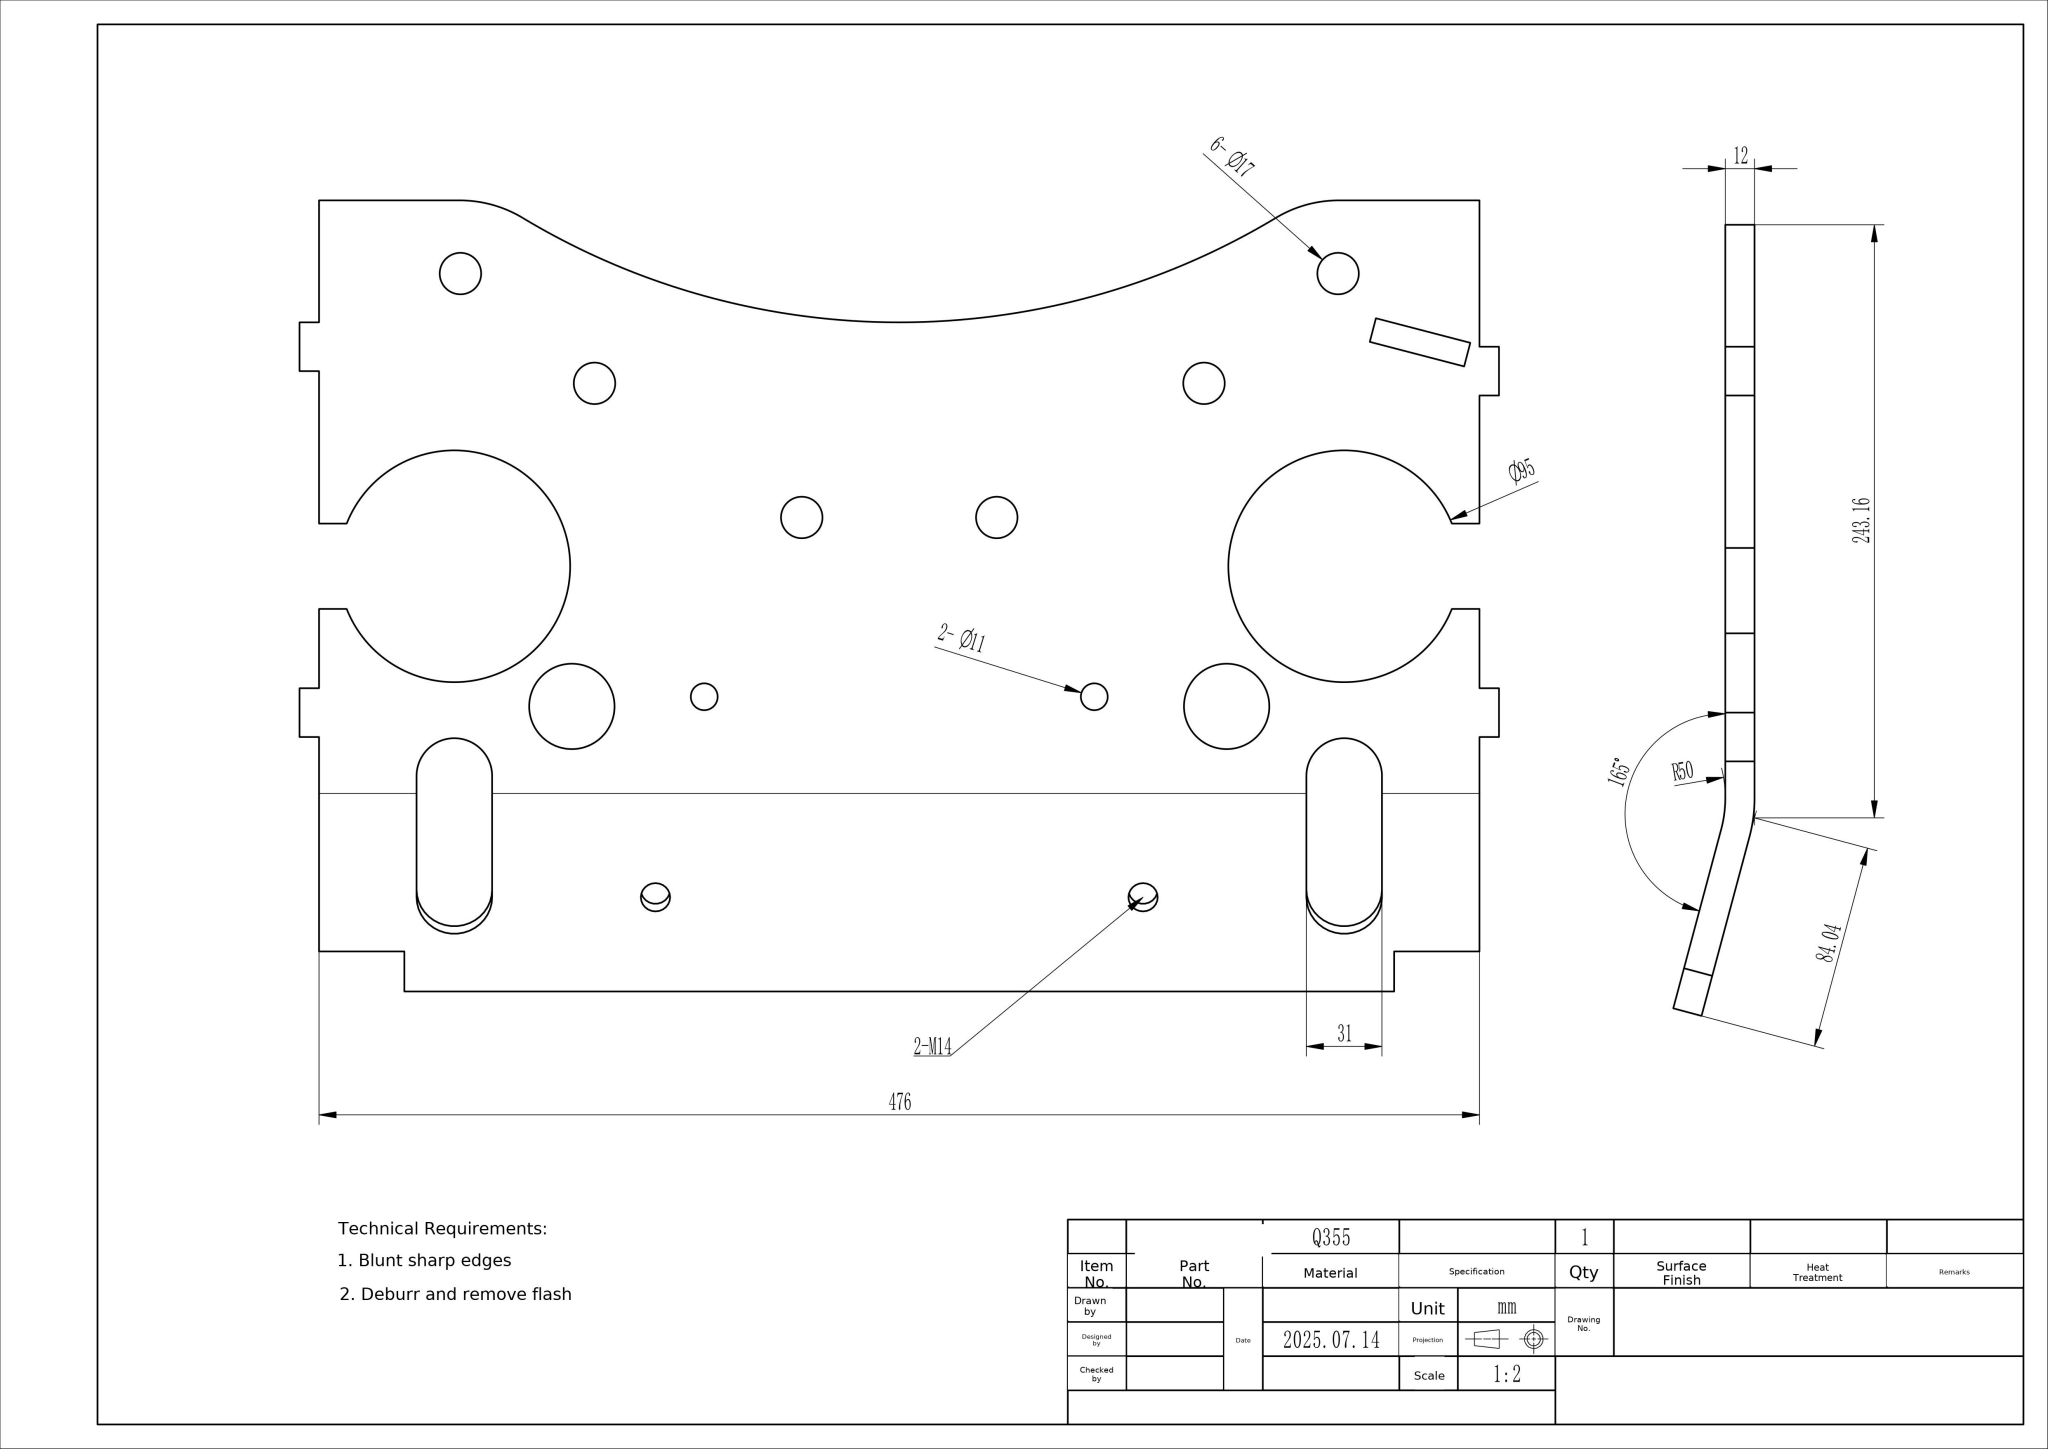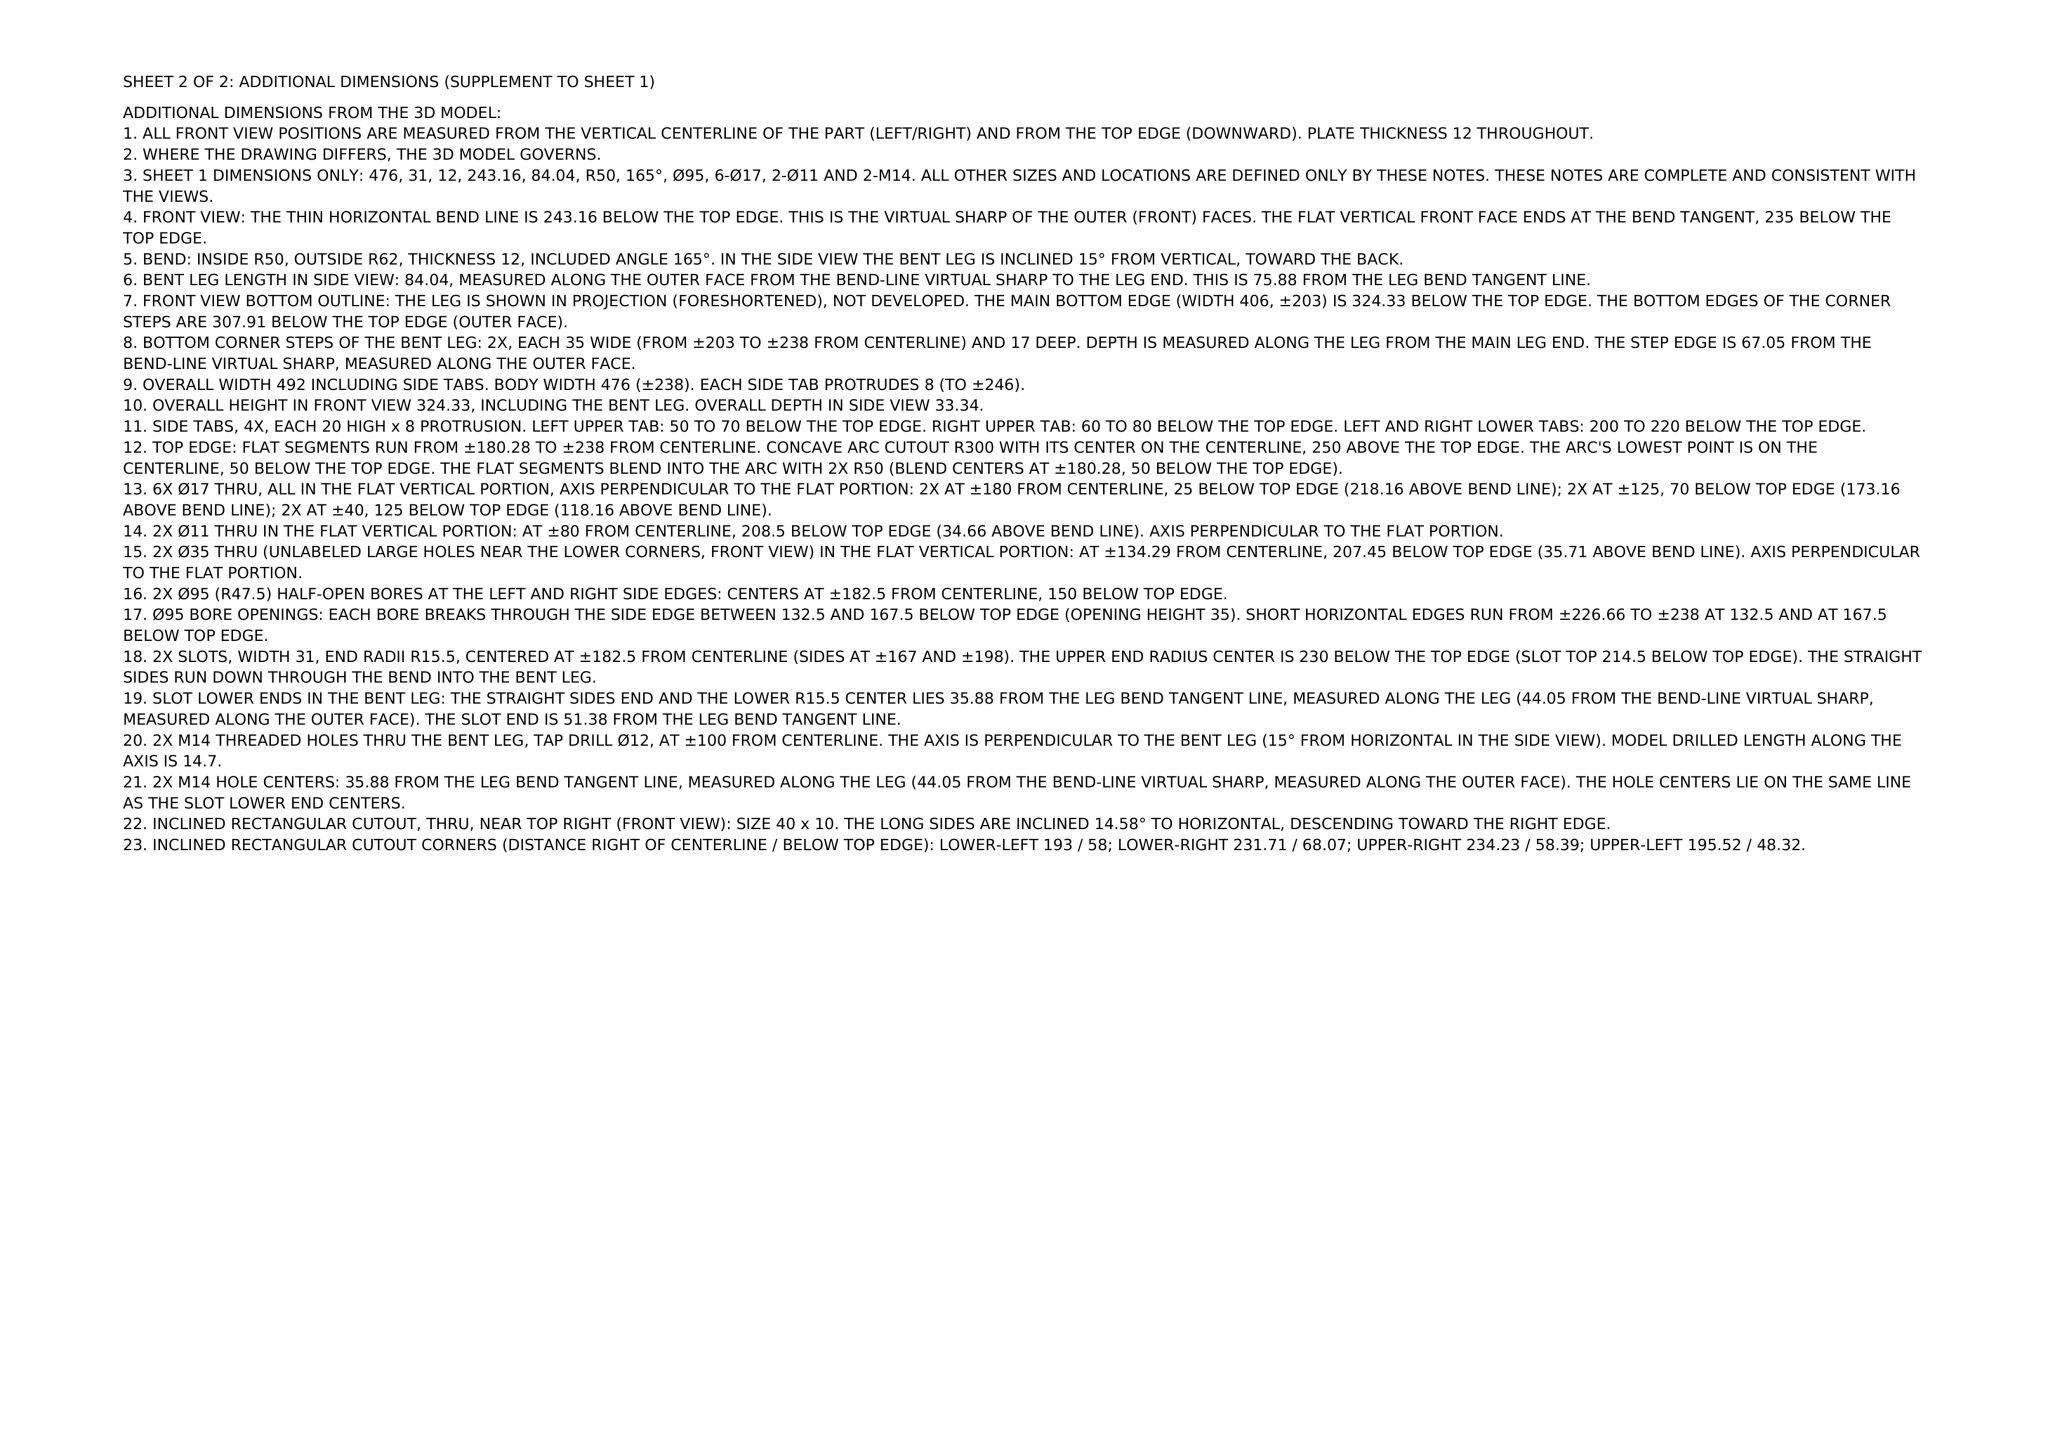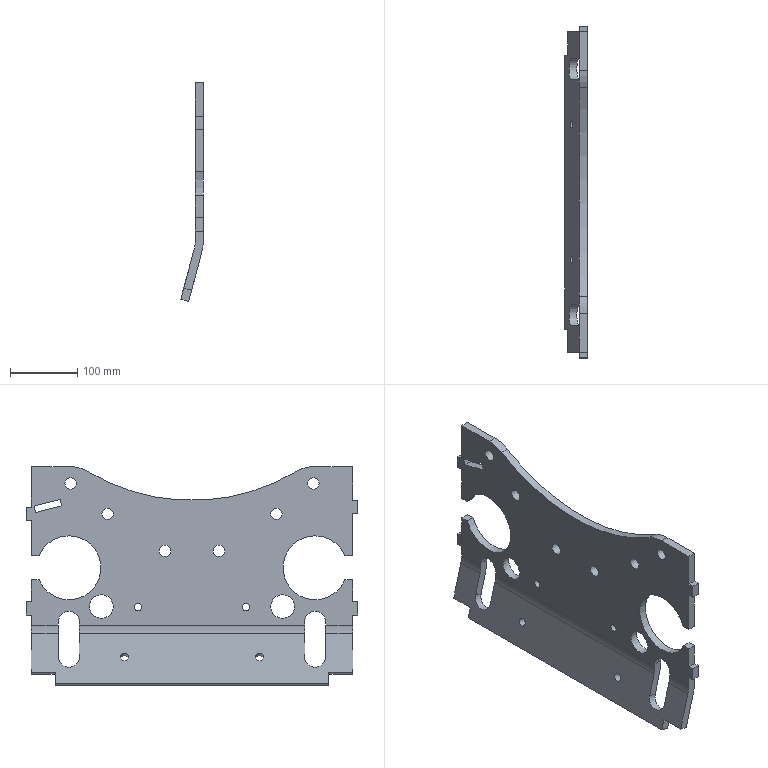Part | NX | mm | 1 solid | 70 faces | box 33.34 x 492 x 324.33 mm | volume 1430943 mm3 | plane 43 | cylinder 27 | commonest cylinder face diameters 17 x6 100 x5 31 x4 124 x3 12 x2 95 x2 11 x2 35 x2